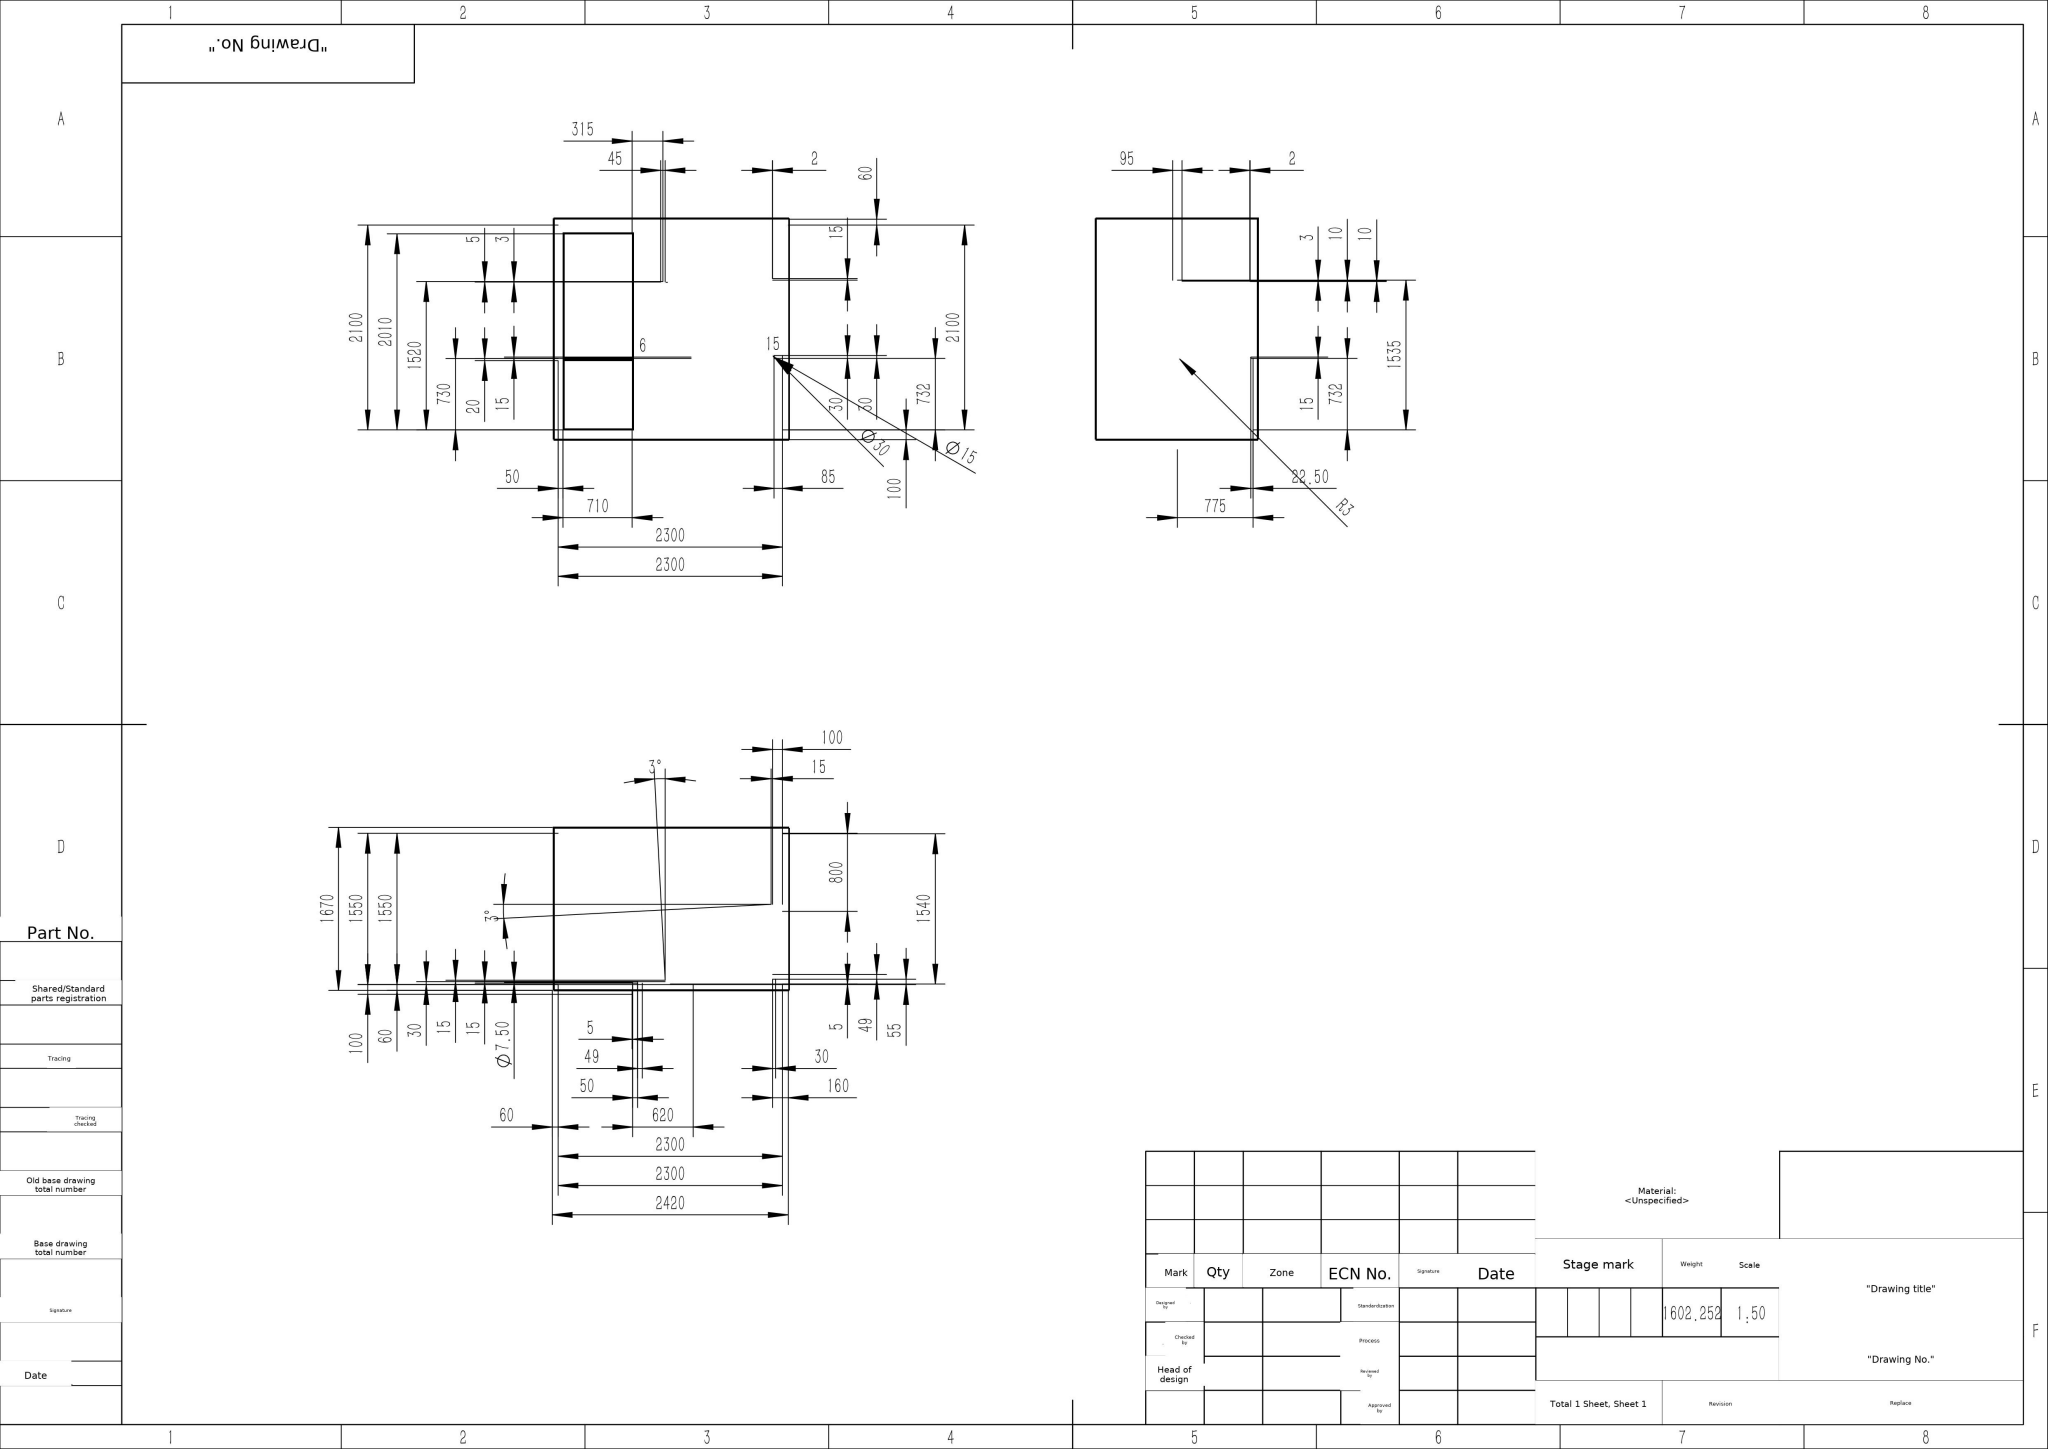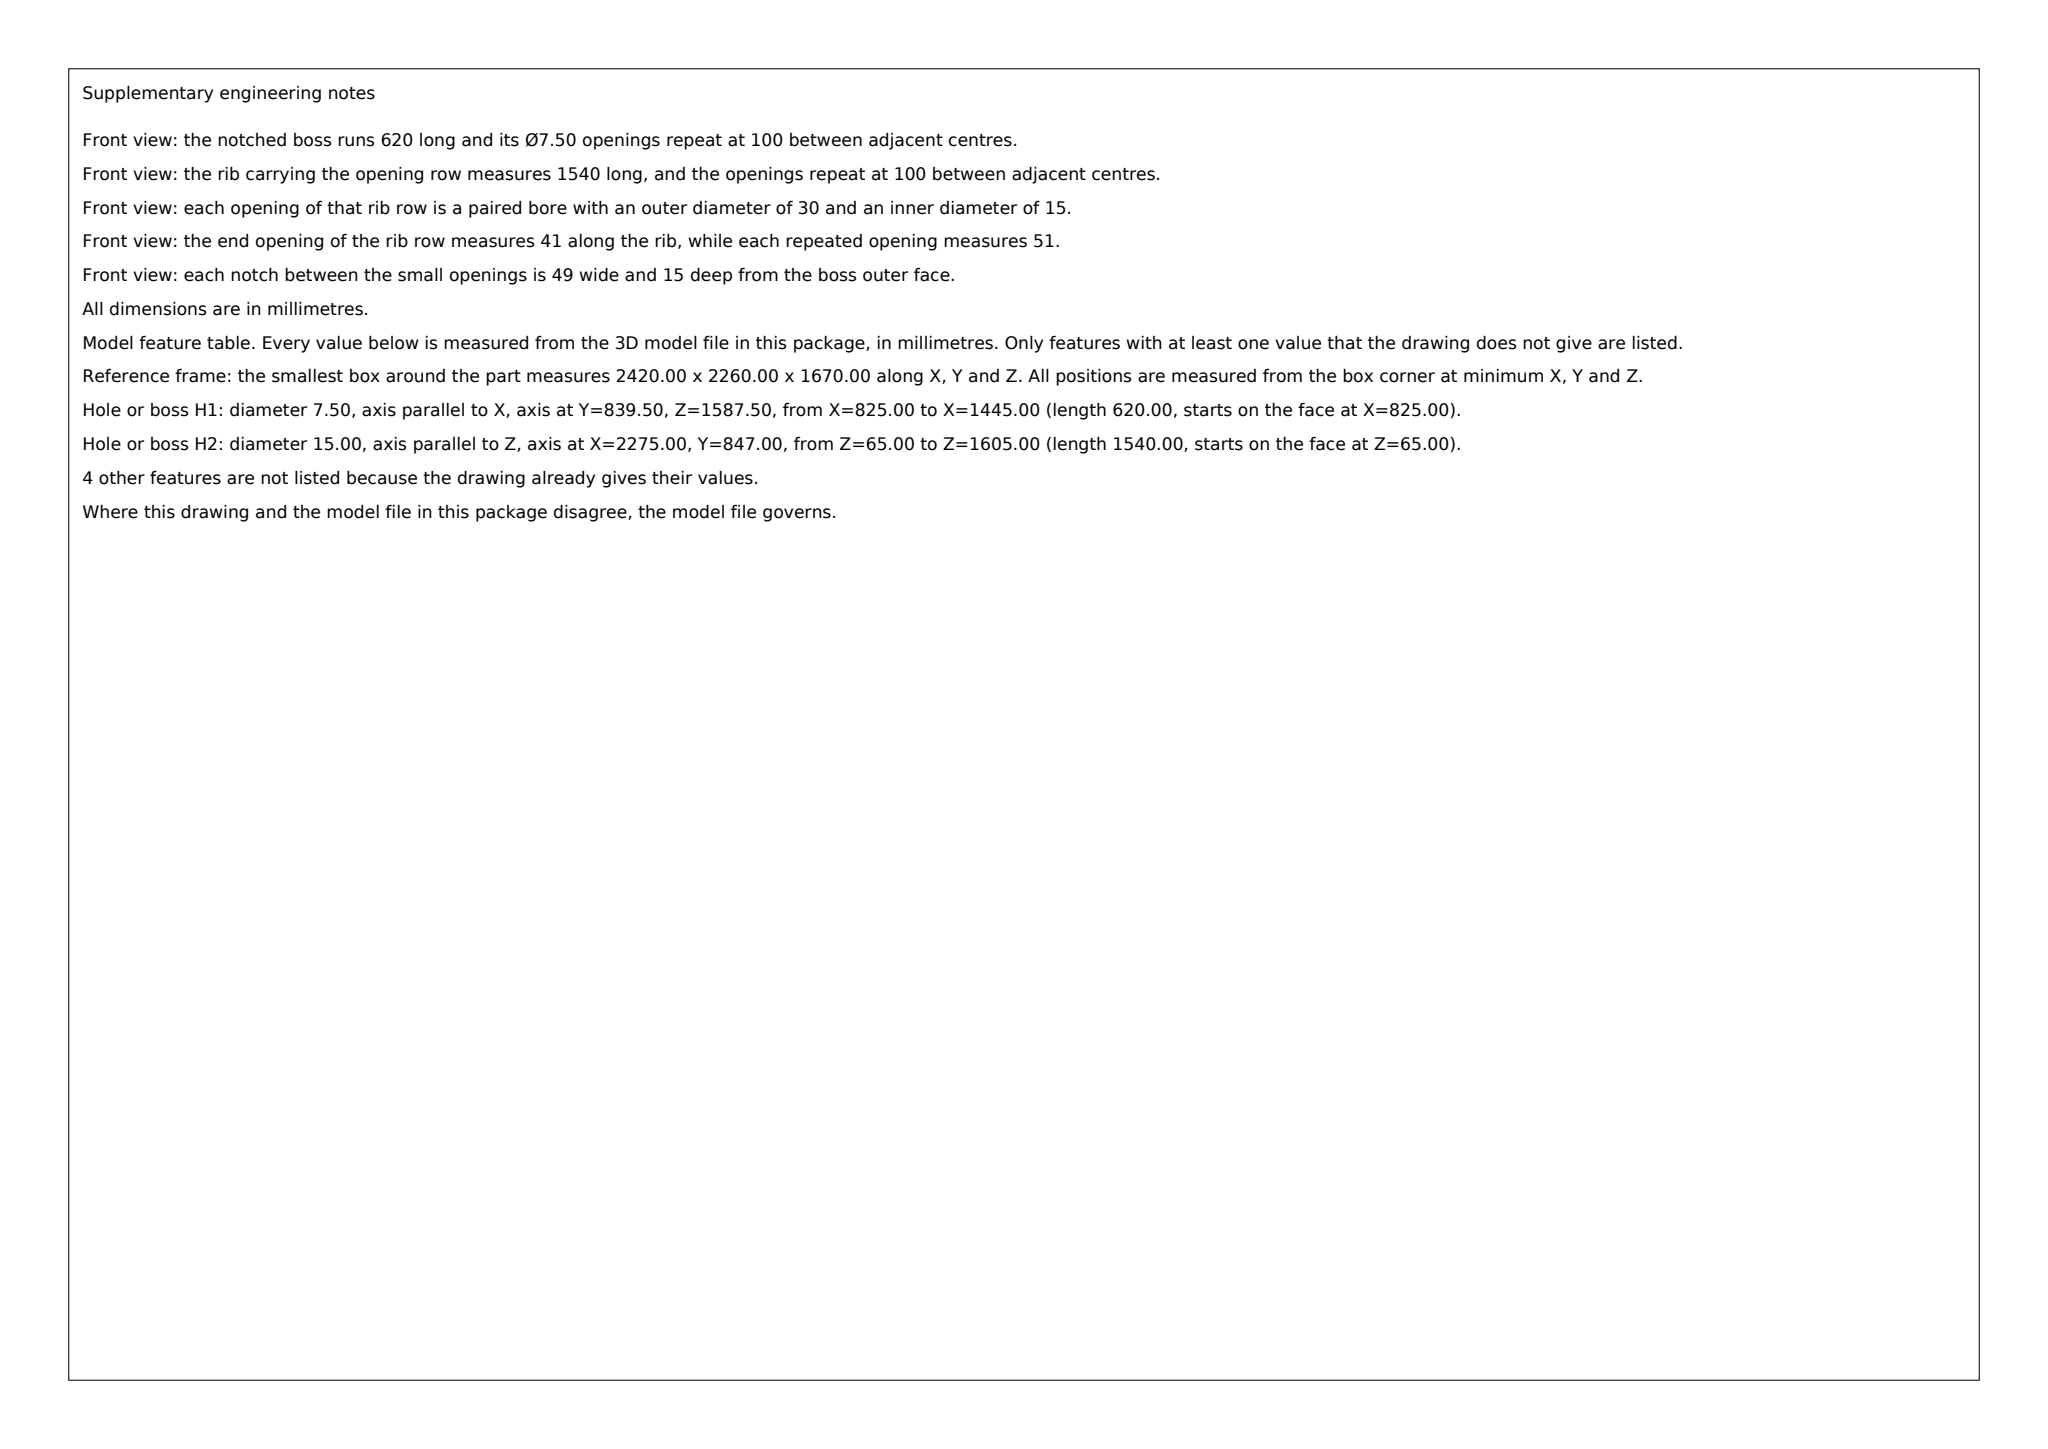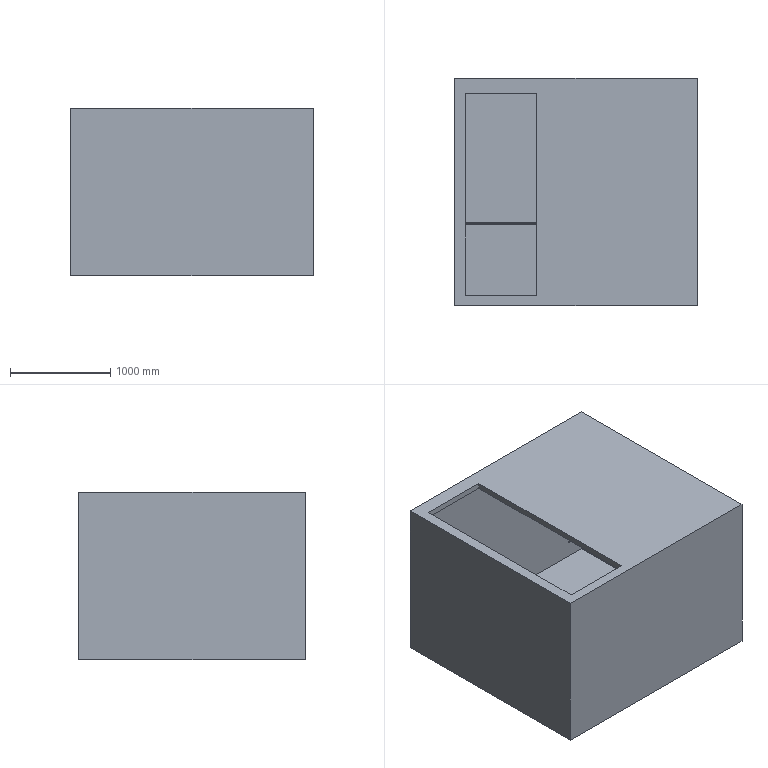Part | SolidWorks | mm | 1 solid | 177 faces | box 2420 x 2260 x 1670 mm | volume 1602252216 mm3 | plane 106 | cylinder 71 | commonest cylinder face diameters 15 x39 30 x16 7.5 x14 6 x2
Drawing notes:
PLAN VIEW: OVERALL DEPTH (Y) 2260 | from the solid: bbox_xyz Y = 2260.0; y-planes 0.0 and 2260.0
16X Ø30 DP 51 / Ø15 THRU, EQ SP 100, 1ST AT 65 FROM BOTTOM | from the solid: Ø30 & Ø15 z-axis cyls at x2275,y847; lengths 41/50/51; z-planes 65-106,155-206...1455-1506,1555-1605 = 100 pitch, 16 places
7X Ø15 DP 51 / Ø7.50 THRU, EQ SP 100, 1ST AT 825 FROM LH END | from the solid: Ø15/Ø7.50 x-axis cyls at y839.5,z1587.5; spans x825-875,924-975,1024-1075,1124-1175,1224-1275,1324-1375,1424-1445
2X Ø6 THRU 2300 LG, 14 C/C ABT Y820, 60 IN FROM EACH END | from the solid: Ø6 x-axis cyls at y813 & y827, z857, length 2300; x-planes 60.0 and 2360.0 (bbox X 2420)
SIDE VIEW: DELETE R3 - ALL EDGES SHARP, NO FILLETS | from the solid: fillet_radii: [] (no fillet faces in model)
2X Ø6 THRU HOLES: AXES 857 ABOVE BOTTOM FACE | from the solid: cylinders dia 6.0 axis x at z=857 (y=813 & 827), bbox z 0-1670